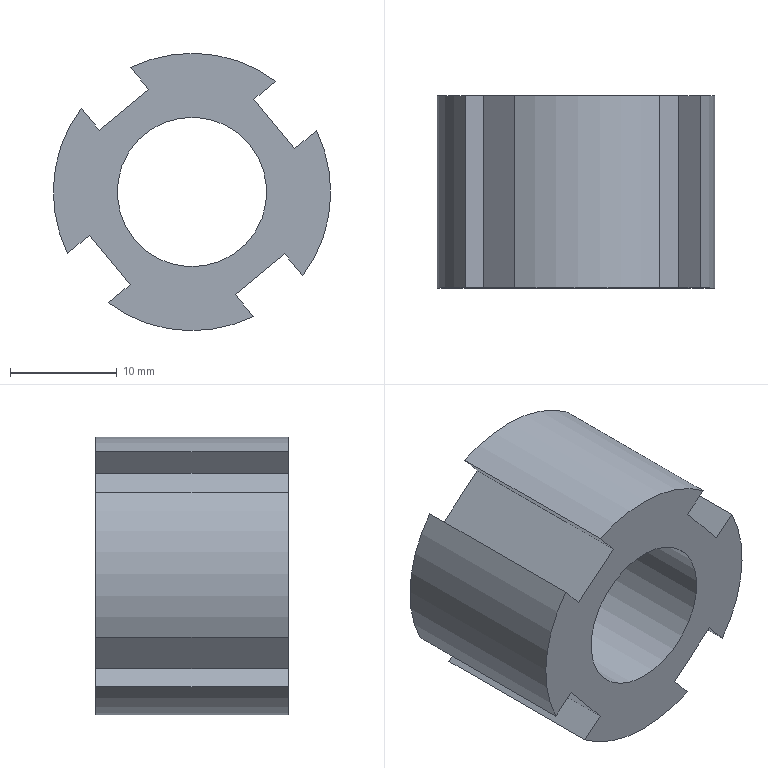Component | SolidWorks | TurntableFixingNut-1 | 1 solid | 20 faces | box 26 x 18 x 26 mm | volume 5540 mm3 | plane 14 | cylinder 6 | commonest cylinder face diameters 26 x4 14 x2
STEP:
#1=COLOUR_RGB('',0.7922,0.8196,0.9333);
#2=FILL_AREA_STYLE_COLOUR('',#1);
#3=FILL_AREA_STYLE('',(#2));
#4=SURFACE_STYLE_FILL_AREA(#3);
#5=SURFACE_SIDE_STYLE('',(#4));
#6=SURFACE_STYLE_USAGE(.BOTH.,#5);
#7=PRESENTATION_STYLE_ASSIGNMENT((#6));
#8=CARTESIAN_POINT('',(-4.58,21.141,7.611));
#9=VERTEX_POINT('',#8);
#10=CARTESIAN_POINT('',(-4.155,21.141,7.963));
#11=VERTEX_POINT('',#10);
#12=CARTESIAN_POINT('',(-4.368,21.141,7.787));
#13=DIRECTION('',(0.,1.,0.));
#14=DIRECTION('',(0.7706,0.,0.6373));
#15=AXIS2_PLACEMENT_3D('',#12,#13,#14);
#16=CIRCLE('',#15,0.2756);
#17=EDGE_CURVE('',#9,#11,#16,.T.);
#18=ORIENTED_EDGE('',*,*,#17,.F.);
#19=CARTESIAN_POINT('',(-4.58,21.85,7.611));
#20=VERTEX_POINT('',#19);
#21=CARTESIAN_POINT('',(-4.58,21.85,7.611));
#22=DIRECTION('',(0.,1.,0.));
#23=VECTOR('',#22,39.37);
#24=LINE('',#21,#23);
#25=EDGE_CURVE('',#9,#20,#24,.T.);
#26=ORIENTED_EDGE('',*,*,#25,.T.);
#27=CARTESIAN_POINT('',(-4.155,21.85,7.963));
#28=VERTEX_POINT('',#27);
#29=CARTESIAN_POINT('',(-4.368,21.85,7.787));
#30=DIRECTION('',(0.,1.,0.));
#31=DIRECTION('',(0.7706,0.,0.6373));
#32=AXIS2_PLACEMENT_3D('',#29,#30,#31);
#33=CIRCLE('',#32,0.2756);
#34=EDGE_CURVE('',#20,#28,#33,.T.);
#35=ORIENTED_EDGE('',*,*,#34,.T.);
#36=CARTESIAN_POINT('',(-4.155,21.85,7.963));
#37=DIRECTION('',(0.,1.,0.));
#38=VECTOR('',#37,39.37);
#39=LINE('',#36,#38);
#40=EDGE_CURVE('',#11,#28,#39,.T.);
#41=ORIENTED_EDGE('',*,*,#40,.F.);
#42=EDGE_LOOP('',(#18,#26,#35,#41));
#43=FACE_OUTER_BOUND('',#42,.T.);
#44=CARTESIAN_POINT('',(-4.368,21.85,7.787));
#45=DIRECTION('',(0.,1.,0.));
#46=DIRECTION('',(0.7706,0.,0.6373));
#47=AXIS2_PLACEMENT_3D('',#44,#45,#46);
#48=CYLINDRICAL_SURFACE('',#47,0.2756);
#49=ADVANCED_FACE('',(#43),#48,.F.);
#50=CARTESIAN_POINT('',(-4.827,21.141,7.561));
#51=VERTEX_POINT('',#50);
#52=CARTESIAN_POINT('',(-4.776,21.141,8.095));
#53=VERTEX_POINT('',#52);
#54=CARTESIAN_POINT('',(-4.368,21.141,7.787));
#55=DIRECTION('',(0.,1.,0.));
#56=DIRECTION('',(0.7706,0.,0.6373));
#57=AXIS2_PLACEMENT_3D('',#54,#55,#56);
#58=CIRCLE('',#57,0.5118);
#59=EDGE_CURVE('',#51,#53,#58,.T.);
#60=ORIENTED_EDGE('',*,*,#59,.T.);
#61=CARTESIAN_POINT('',(-4.776,21.85,8.095));
#62=VERTEX_POINT('',#61);
#63=CARTESIAN_POINT('',(-4.776,21.85,8.095));
#64=DIRECTION('',(0.,-1.,0.));
#65=VECTOR('',#64,39.37);
#66=LINE('',#63,#65);
#67=EDGE_CURVE('',#62,#53,#66,.T.);
#68=ORIENTED_EDGE('',*,*,#67,.F.);
#69=CARTESIAN_POINT('',(-4.827,21.85,7.561));
#70=VERTEX_POINT('',#69);
#71=CARTESIAN_POINT('',(-4.368,21.85,7.787));
#72=DIRECTION('',(0.,1.,0.));
#73=DIRECTION('',(0.7706,0.,0.6373));
#74=AXIS2_PLACEMENT_3D('',#71,#72,#73);
#75=CIRCLE('',#74,0.5118);
#76=EDGE_CURVE('',#70,#62,#75,.T.);
#77=ORIENTED_EDGE('',*,*,#76,.F.);
#78=CARTESIAN_POINT('',(-4.827,21.85,7.561));
#79=DIRECTION('',(0.,-1.,0.));
#80=VECTOR('',#79,39.37);
#81=LINE('',#78,#80);
#82=EDGE_CURVE('',#70,#51,#81,.T.);
#83=ORIENTED_EDGE('',*,*,#82,.T.);
#84=EDGE_LOOP('',(#60,#68,#77,#83));
#85=FACE_OUTER_BOUND('',#84,.T.);
#86=CARTESIAN_POINT('',(-4.368,21.85,7.787));
#87=DIRECTION('',(0.,-1.,0.));
#88=DIRECTION('',(-0.7706,0.,-0.6373));
#89=AXIS2_PLACEMENT_3D('',#86,#87,#88);
#90=CYLINDRICAL_SURFACE('',#89,0.5118);
#91=ADVANCED_FACE('',(#85),#90,.T.);
#92=CARTESIAN_POINT('',(-4.71,21.141,8.015));
#93=VERTEX_POINT('',#92);
#94=CARTESIAN_POINT('',(-4.776,21.141,8.095));
#95=DIRECTION('',(0.6373,0.,-0.7706));
#96=VECTOR('',#95,39.37);
#97=LINE('',#94,#96);
#98=EDGE_CURVE('',#53,#93,#97,.T.);
#99=ORIENTED_EDGE('',*,*,#98,.T.);
#100=CARTESIAN_POINT('',(-4.71,21.85,8.015));
#101=VERTEX_POINT('',#100);
#102=CARTESIAN_POINT('',(-4.71,21.85,8.015));
#103=DIRECTION('',(0.,-1.,0.));
#104=VECTOR('',#103,39.37);
#105=LINE('',#102,#104);
#106=EDGE_CURVE('',#101,#93,#105,.T.);
#107=ORIENTED_EDGE('',*,*,#106,.F.);
#108=CARTESIAN_POINT('',(-4.776,21.85,8.095));
#109=DIRECTION('',(0.6373,0.,-0.7706));
#110=VECTOR('',#109,39.37);
#111=LINE('',#108,#110);
#112=EDGE_CURVE('',#62,#101,#111,.T.);
#113=ORIENTED_EDGE('',*,*,#112,.F.);
#114=ORIENTED_EDGE('',*,*,#67,.T.);
#115=EDGE_LOOP('',(#99,#107,#113,#114));
#116=FACE_OUTER_BOUND('',#115,.T.);
#117=CARTESIAN_POINT('',(-4.776,21.85,8.095));
#118=DIRECTION('',(-0.7706,0.,-0.6373));
#119=DIRECTION('',(-0.6373,0.,0.7706));
#120=AXIS2_PLACEMENT_3D('',#117,#118,#119);
#121=PLANE('',#120);
#122=ADVANCED_FACE('',(#116),#121,.F.);
#123=CARTESIAN_POINT('',(-4.528,21.141,8.166));
#124=VERTEX_POINT('',#123);
#125=CARTESIAN_POINT('',(-4.528,21.141,8.166));
#126=DIRECTION('',(0.7706,0.,0.6373));
#127=VECTOR('',#126,39.37);
#128=LINE('',#125,#127);
#129=EDGE_CURVE('',#93,#124,#128,.T.);
#130=ORIENTED_EDGE('',*,*,#129,.T.);
#131=CARTESIAN_POINT('',(-4.528,21.85,8.166));
#132=VERTEX_POINT('',#131);
#133=CARTESIAN_POINT('',(-4.528,21.85,8.166));
#134=DIRECTION('',(0.,-1.,0.));
#135=VECTOR('',#134,39.37);
#136=LINE('',#133,#135);
#137=EDGE_CURVE('',#132,#124,#136,.T.);
#138=ORIENTED_EDGE('',*,*,#137,.F.);
#139=CARTESIAN_POINT('',(-4.528,21.85,8.166));
#140=DIRECTION('',(0.7706,0.,0.6373));
#141=VECTOR('',#140,39.37);
#142=LINE('',#139,#141);
#143=EDGE_CURVE('',#101,#132,#142,.T.);
#144=ORIENTED_EDGE('',*,*,#143,.F.);
#145=ORIENTED_EDGE('',*,*,#106,.T.);
#146=EDGE_LOOP('',(#130,#138,#144,#145));
#147=FACE_OUTER_BOUND('',#146,.T.);
#148=CARTESIAN_POINT('',(-4.528,21.85,8.166));
#149=DIRECTION('',(0.6373,0.,-0.7706));
#150=DIRECTION('',(-0.7706,0.,-0.6373));
#151=AXIS2_PLACEMENT_3D('',#148,#149,#150);
#152=PLANE('',#151);
#153=ADVANCED_FACE('',(#147),#152,.F.);
#154=CARTESIAN_POINT('',(-4.594,21.141,8.246));
#155=VERTEX_POINT('',#154);
#156=CARTESIAN_POINT('',(-4.594,21.141,8.246));
#157=DIRECTION('',(-0.6373,0.,0.7706));
#158=VECTOR('',#157,39.37);
#159=LINE('',#156,#158);
#160=EDGE_CURVE('',#124,#155,#159,.T.);
#161=ORIENTED_EDGE('',*,*,#160,.T.);
#162=CARTESIAN_POINT('',(-4.594,21.85,8.246));
#163=VERTEX_POINT('',#162);
#164=CARTESIAN_POINT('',(-4.594,21.85,8.246));
#165=DIRECTION('',(0.,-1.,0.));
#166=VECTOR('',#165,39.37);
#167=LINE('',#164,#166);
#168=EDGE_CURVE('',#163,#155,#167,.T.);
#169=ORIENTED_EDGE('',*,*,#168,.F.);
#170=CARTESIAN_POINT('',(-4.594,21.85,8.246));
#171=DIRECTION('',(-0.6373,0.,0.7706));
#172=VECTOR('',#171,39.37);
#173=LINE('',#170,#172);
#174=EDGE_CURVE('',#132,#163,#173,.T.);
#175=ORIENTED_EDGE('',*,*,#174,.F.);
#176=ORIENTED_EDGE('',*,*,#137,.T.);
#177=EDGE_LOOP('',(#161,#169,#175,#176));
#178=FACE_OUTER_BOUND('',#177,.T.);
#179=CARTESIAN_POINT('',(-4.594,21.85,8.246));
#180=DIRECTION('',(0.7706,0.,0.6373));
#181=DIRECTION('',(0.6373,0.,-0.7706));
#182=AXIS2_PLACEMENT_3D('',#179,#180,#181);
#183=PLANE('',#182);
#184=ADVANCED_FACE('',(#178),#183,.F.);
#185=CARTESIAN_POINT('',(-4.059,21.141,8.195));
#186=VERTEX_POINT('',#185);
#187=CARTESIAN_POINT('',(-4.368,21.141,7.787));
#188=DIRECTION('',(0.,1.,0.));
#189=DIRECTION('',(0.7706,0.,0.6373));
#190=AXIS2_PLACEMENT_3D('',#187,#188,#189);
#191=CIRCLE('',#190,0.5118);
#192=EDGE_CURVE('',#155,#186,#191,.T.);
#193=ORIENTED_EDGE('',*,*,#192,.T.);
#194=CARTESIAN_POINT('',(-4.059,21.85,8.195));
#195=VERTEX_POINT('',#194);
#196=CARTESIAN_POINT('',(-4.059,21.85,8.195));
#197=DIRECTION('',(0.,-1.,0.));
#198=VECTOR('',#197,39.37);
#199=LINE('',#196,#198);
#200=EDGE_CURVE('',#195,#186,#199,.T.);
#201=ORIENTED_EDGE('',*,*,#200,.F.);
#202=CARTESIAN_POINT('',(-4.368,21.85,7.787));
#203=DIRECTION('',(0.,1.,0.));
#204=DIRECTION('',(0.7706,0.,0.6373));
#205=AXIS2_PLACEMENT_3D('',#202,#203,#204);
#206=CIRCLE('',#205,0.5118);
#207=EDGE_CURVE('',#163,#195,#206,.T.);
#208=ORIENTED_EDGE('',*,*,#207,.F.);
#209=ORIENTED_EDGE('',*,*,#168,.T.);
#210=EDGE_LOOP('',(#193,#201,#208,#209));
#211=FACE_OUTER_BOUND('',#210,.T.);
#212=CARTESIAN_POINT('',(-4.368,21.85,7.787));
#213=DIRECTION('',(0.,-1.,0.));
#214=DIRECTION('',(-0.7706,0.,-0.6373));
#215=AXIS2_PLACEMENT_3D('',#212,#213,#214);
#216=CYLINDRICAL_SURFACE('',#215,0.5118);
#217=ADVANCED_FACE('',(#211),#216,.T.);
#218=CARTESIAN_POINT('',(-4.14,21.141,8.129));
#219=VERTEX_POINT('',#218);
#220=CARTESIAN_POINT('',(-4.059,21.141,8.195));
#221=DIRECTION('',(-0.7706,0.,-0.6373));
#222=VECTOR('',#221,39.37);
#223=LINE('',#220,#222);
#224=EDGE_CURVE('',#186,#219,#223,.T.);
#225=ORIENTED_EDGE('',*,*,#224,.T.);
#226=CARTESIAN_POINT('',(-4.14,21.85,8.129));
#227=VERTEX_POINT('',#226);
#228=CARTESIAN_POINT('',(-4.14,21.85,8.129));
#229=DIRECTION('',(0.,-1.,0.));
#230=VECTOR('',#229,39.37);
#231=LINE('',#228,#230);
#232=EDGE_CURVE('',#227,#219,#231,.T.);
#233=ORIENTED_EDGE('',*,*,#232,.F.);
#234=CARTESIAN_POINT('',(-4.059,21.85,8.195));
#235=DIRECTION('',(-0.7706,0.,-0.6373));
#236=VECTOR('',#235,39.37);
#237=LINE('',#234,#236);
#238=EDGE_CURVE('',#195,#227,#237,.T.);
#239=ORIENTED_EDGE('',*,*,#238,.F.);
#240=ORIENTED_EDGE('',*,*,#200,.T.);
#241=EDGE_LOOP('',(#225,#233,#239,#240));
#242=FACE_OUTER_BOUND('',#241,.T.);
#243=CARTESIAN_POINT('',(-4.059,21.85,8.195));
#244=DIRECTION('',(-0.6373,0.,0.7706));
#245=DIRECTION('',(0.7706,0.,0.6373));
#246=AXIS2_PLACEMENT_3D('',#243,#244,#245);
#247=PLANE('',#246);
#248=ADVANCED_FACE('',(#242),#247,.F.);
#249=CARTESIAN_POINT('',(-3.989,21.141,7.947));
#250=VERTEX_POINT('',#249);
#251=CARTESIAN_POINT('',(-3.989,21.141,7.947));
#252=DIRECTION('',(0.6373,0.,-0.7706));
#253=VECTOR('',#252,39.37);
#254=LINE('',#251,#253);
#255=EDGE_CURVE('',#219,#250,#254,.T.);
#256=ORIENTED_EDGE('',*,*,#255,.T.);
#257=CARTESIAN_POINT('',(-3.989,21.85,7.947));
#258=VERTEX_POINT('',#257);
#259=CARTESIAN_POINT('',(-3.989,21.85,7.947));
#260=DIRECTION('',(0.,-1.,0.));
#261=VECTOR('',#260,39.37);
#262=LINE('',#259,#261);
#263=EDGE_CURVE('',#258,#250,#262,.T.);
#264=ORIENTED_EDGE('',*,*,#263,.F.);
#265=CARTESIAN_POINT('',(-3.989,21.85,7.947));
#266=DIRECTION('',(0.6373,0.,-0.7706));
#267=VECTOR('',#266,39.37);
#268=LINE('',#265,#267);
#269=EDGE_CURVE('',#227,#258,#268,.T.);
#270=ORIENTED_EDGE('',*,*,#269,.F.);
#271=ORIENTED_EDGE('',*,*,#232,.T.);
#272=EDGE_LOOP('',(#256,#264,#270,#271));
#273=FACE_OUTER_BOUND('',#272,.T.);
#274=CARTESIAN_POINT('',(-3.989,21.85,7.947));
#275=DIRECTION('',(-0.7706,0.,-0.6373));
#276=DIRECTION('',(-0.6373,0.,0.7706));
#277=AXIS2_PLACEMENT_3D('',#274,#275,#276);
#278=PLANE('',#277);
#279=ADVANCED_FACE('',(#273),#278,.F.);
#280=CARTESIAN_POINT('',(-3.909,21.141,8.013));
#281=VERTEX_POINT('',#280);
#282=CARTESIAN_POINT('',(-3.909,21.141,8.013));
#283=DIRECTION('',(0.7706,0.,0.6373));
#284=VECTOR('',#283,39.37);
#285=LINE('',#282,#284);
#286=EDGE_CURVE('',#250,#281,#285,.T.);
#287=ORIENTED_EDGE('',*,*,#286,.T.);
#288=CARTESIAN_POINT('',(-3.909,21.85,8.013));
#289=VERTEX_POINT('',#288);
#290=CARTESIAN_POINT('',(-3.909,21.85,8.013));
#291=DIRECTION('',(0.,-1.,0.));
#292=VECTOR('',#291,39.37);
#293=LINE('',#290,#292);
#294=EDGE_CURVE('',#289,#281,#293,.T.);
#295=ORIENTED_EDGE('',*,*,#294,.F.);
#296=CARTESIAN_POINT('',(-3.909,21.85,8.013));
#297=DIRECTION('',(0.7706,0.,0.6373));
#298=VECTOR('',#297,39.37);
#299=LINE('',#296,#298);
#300=EDGE_CURVE('',#258,#289,#299,.T.);
#301=ORIENTED_EDGE('',*,*,#300,.F.);
#302=ORIENTED_EDGE('',*,*,#263,.T.);
#303=EDGE_LOOP('',(#287,#295,#301,#302));
#304=FACE_OUTER_BOUND('',#303,.T.);
#305=CARTESIAN_POINT('',(-3.909,21.85,8.013));
#306=DIRECTION('',(0.6373,0.,-0.7706));
#307=DIRECTION('',(-0.7706,0.,-0.6373));
#308=AXIS2_PLACEMENT_3D('',#305,#306,#307);
#309=PLANE('',#308);
#310=ADVANCED_FACE('',(#304),#309,.F.);
#311=CARTESIAN_POINT('',(-3.959,21.141,7.478));
#312=VERTEX_POINT('',#311);
#313=CARTESIAN_POINT('',(-4.368,21.141,7.787));
#314=DIRECTION('',(0.,1.,0.));
#315=DIRECTION('',(0.7706,0.,0.6373));
#316=AXIS2_PLACEMENT_3D('',#313,#314,#315);
#317=CIRCLE('',#316,0.5118);
#318=EDGE_CURVE('',#281,#312,#317,.T.);
#319=ORIENTED_EDGE('',*,*,#318,.T.);
#320=CARTESIAN_POINT('',(-3.959,21.85,7.478));
#321=VERTEX_POINT('',#320);
#322=CARTESIAN_POINT('',(-3.959,21.85,7.478));
#323=DIRECTION('',(0.,-1.,0.));
#324=VECTOR('',#323,39.37);
#325=LINE('',#322,#324);
#326=EDGE_CURVE('',#321,#312,#325,.T.);
#327=ORIENTED_EDGE('',*,*,#326,.F.);
#328=CARTESIAN_POINT('',(-4.368,21.85,7.787));
#329=DIRECTION('',(0.,1.,0.));
#330=DIRECTION('',(0.7706,0.,0.6373));
#331=AXIS2_PLACEMENT_3D('',#328,#329,#330);
#332=CIRCLE('',#331,0.5118);
#333=EDGE_CURVE('',#289,#321,#332,.T.);
#334=ORIENTED_EDGE('',*,*,#333,.F.);
#335=ORIENTED_EDGE('',*,*,#294,.T.);
#336=EDGE_LOOP('',(#319,#327,#334,#335));
#337=FACE_OUTER_BOUND('',#336,.T.);
#338=CARTESIAN_POINT('',(-4.368,21.85,7.787));
#339=DIRECTION('',(0.,-1.,0.));
#340=DIRECTION('',(-0.7706,0.,-0.6373));
#341=AXIS2_PLACEMENT_3D('',#338,#339,#340);
#342=CYLINDRICAL_SURFACE('',#341,0.5118);
#343=ADVANCED_FACE('',(#337),#342,.T.);
#344=CARTESIAN_POINT('',(-4.026,21.141,7.559));
#345=VERTEX_POINT('',#344);
#346=CARTESIAN_POINT('',(-3.959,21.141,7.478));
#347=DIRECTION('',(-0.6373,0.,0.7706));
#348=VECTOR('',#347,39.37);
#349=LINE('',#346,#348);
#350=EDGE_CURVE('',#312,#345,#349,.T.);
#351=ORIENTED_EDGE('',*,*,#350,.T.);
#352=CARTESIAN_POINT('',(-4.026,21.85,7.559));
#353=VERTEX_POINT('',#352);
#354=CARTESIAN_POINT('',(-4.026,21.85,7.559));
#355=DIRECTION('',(0.,-1.,0.));
#356=VECTOR('',#355,39.37);
#357=LINE('',#354,#356);
#358=EDGE_CURVE('',#353,#345,#357,.T.);
#359=ORIENTED_EDGE('',*,*,#358,.F.);
#360=CARTESIAN_POINT('',(-3.959,21.85,7.478));
#361=DIRECTION('',(-0.6373,0.,0.7706));
#362=VECTOR('',#361,39.37);
#363=LINE('',#360,#362);
#364=EDGE_CURVE('',#321,#353,#363,.T.);
#365=ORIENTED_EDGE('',*,*,#364,.F.);
#366=ORIENTED_EDGE('',*,*,#326,.T.);
#367=EDGE_LOOP('',(#351,#359,#365,#366));
#368=FACE_OUTER_BOUND('',#367,.T.);
#369=CARTESIAN_POINT('',(-3.959,21.85,7.478));
#370=DIRECTION('',(0.7706,0.,0.6373));
#371=DIRECTION('',(0.6373,0.,-0.7706));
#372=AXIS2_PLACEMENT_3D('',#369,#370,#371);
#373=PLANE('',#372);
#374=ADVANCED_FACE('',(#368),#373,.F.);
#375=CARTESIAN_POINT('',(-4.208,21.141,7.408));
#376=VERTEX_POINT('',#375);
#377=CARTESIAN_POINT('',(-4.208,21.141,7.408));
#378=DIRECTION('',(-0.7706,0.,-0.6373));
#379=VECTOR('',#378,39.37);
#380=LINE('',#377,#379);
#381=EDGE_CURVE('',#345,#376,#380,.T.);
#382=ORIENTED_EDGE('',*,*,#381,.T.);
#383=CARTESIAN_POINT('',(-4.208,21.85,7.408));
#384=VERTEX_POINT('',#383);
#385=CARTESIAN_POINT('',(-4.208,21.85,7.408));
#386=DIRECTION('',(0.,-1.,0.));
#387=VECTOR('',#386,39.37);
#388=LINE('',#385,#387);
#389=EDGE_CURVE('',#384,#376,#388,.T.);
#390=ORIENTED_EDGE('',*,*,#389,.F.);
#391=CARTESIAN_POINT('',(-4.208,21.85,7.408));
#392=DIRECTION('',(-0.7706,0.,-0.6373));
#393=VECTOR('',#392,39.37);
#394=LINE('',#391,#393);
#395=EDGE_CURVE('',#353,#384,#394,.T.);
#396=ORIENTED_EDGE('',*,*,#395,.F.);
#397=ORIENTED_EDGE('',*,*,#358,.T.);
#398=EDGE_LOOP('',(#382,#390,#396,#397));
#399=FACE_OUTER_BOUND('',#398,.T.);
#400=CARTESIAN_POINT('',(-4.208,21.85,7.408));
#401=DIRECTION('',(-0.6373,0.,0.7706));
#402=DIRECTION('',(0.7706,0.,0.6373));
#403=AXIS2_PLACEMENT_3D('',#400,#401,#402);
#404=PLANE('',#403);
#405=ADVANCED_FACE('',(#399),#404,.F.);
#406=CARTESIAN_POINT('',(-4.142,21.141,7.328));
#407=VERTEX_POINT('',#406);
#408=CARTESIAN_POINT('',(-4.142,21.141,7.328));
#409=DIRECTION('',(0.6373,0.,-0.7706));
#410=VECTOR('',#409,39.37);
#411=LINE('',#408,#410);
#412=EDGE_CURVE('',#376,#407,#411,.T.);
#413=ORIENTED_EDGE('',*,*,#412,.T.);
#414=CARTESIAN_POINT('',(-4.142,21.85,7.328));
#415=VERTEX_POINT('',#414);
#416=CARTESIAN_POINT('',(-4.142,21.85,7.328));
#417=DIRECTION('',(0.,-1.,0.));
#418=VECTOR('',#417,39.37);
#419=LINE('',#416,#418);
#420=EDGE_CURVE('',#415,#407,#419,.T.);
#421=ORIENTED_EDGE('',*,*,#420,.F.);
#422=CARTESIAN_POINT('',(-4.142,21.85,7.328));
#423=DIRECTION('',(0.6373,0.,-0.7706));
#424=VECTOR('',#423,39.37);
#425=LINE('',#422,#424);
#426=EDGE_CURVE('',#384,#415,#425,.T.);
#427=ORIENTED_EDGE('',*,*,#426,.F.);
#428=ORIENTED_EDGE('',*,*,#389,.T.);
#429=EDGE_LOOP('',(#413,#421,#427,#428));
#430=FACE_OUTER_BOUND('',#429,.T.);
#431=CARTESIAN_POINT('',(-4.142,21.85,7.328));
#432=DIRECTION('',(-0.7706,0.,-0.6373));
#433=DIRECTION('',(-0.6373,0.,0.7706));
#434=AXIS2_PLACEMENT_3D('',#431,#432,#433);
#435=PLANE('',#434);
#436=ADVANCED_FACE('',(#430),#435,.F.);
#437=CARTESIAN_POINT('',(-4.676,21.141,7.379));
#438=VERTEX_POINT('',#437);
#439=CARTESIAN_POINT('',(-4.368,21.141,7.787));
#440=DIRECTION('',(0.,1.,0.));
#441=DIRECTION('',(0.7706,0.,0.6373));
#442=AXIS2_PLACEMENT_3D('',#439,#440,#441);
#443=CIRCLE('',#442,0.5118);
#444=EDGE_CURVE('',#407,#438,#443,.T.);
#445=ORIENTED_EDGE('',*,*,#444,.T.);
#446=CARTESIAN_POINT('',(-4.676,21.85,7.379));
#447=VERTEX_POINT('',#446);
#448=CARTESIAN_POINT('',(-4.676,21.85,7.379));
#449=DIRECTION('',(0.,-1.,0.));
#450=VECTOR('',#449,39.37);
#451=LINE('',#448,#450);
#452=EDGE_CURVE('',#447,#438,#451,.T.);
#453=ORIENTED_EDGE('',*,*,#452,.F.);
#454=CARTESIAN_POINT('',(-4.368,21.85,7.787));
#455=DIRECTION('',(0.,1.,0.));
#456=DIRECTION('',(0.7706,0.,0.6373));
#457=AXIS2_PLACEMENT_3D('',#454,#455,#456);
#458=CIRCLE('',#457,0.5118);
#459=EDGE_CURVE('',#415,#447,#458,.T.);
#460=ORIENTED_EDGE('',*,*,#459,.F.);
#461=ORIENTED_EDGE('',*,*,#420,.T.);
#462=EDGE_LOOP('',(#445,#453,#460,#461));
#463=FACE_OUTER_BOUND('',#462,.T.);
#464=CARTESIAN_POINT('',(-4.368,21.85,7.787));
#465=DIRECTION('',(0.,-1.,0.));
#466=DIRECTION('',(-0.7706,0.,-0.6373));
#467=AXIS2_PLACEMENT_3D('',#464,#465,#466);
#468=CYLINDRICAL_SURFACE('',#467,0.5118);
#469=ADVANCED_FACE('',(#463),#468,.T.);
#470=CARTESIAN_POINT('',(-4.596,21.141,7.445));
#471=VERTEX_POINT('',#470);
#472=CARTESIAN_POINT('',(-4.676,21.141,7.379));
#473=DIRECTION('',(0.7706,0.,0.6373));
#474=VECTOR('',#473,39.37);
#475=LINE('',#472,#474);
#476=EDGE_CURVE('',#438,#471,#475,.T.);
#477=ORIENTED_EDGE('',*,*,#476,.T.);
#478=CARTESIAN_POINT('',(-4.596,21.85,7.445));
#479=VERTEX_POINT('',#478);
#480=CARTESIAN_POINT('',(-4.596,21.85,7.445));
#481=DIRECTION('',(0.,-1.,0.));
#482=VECTOR('',#481,39.37);
#483=LINE('',#480,#482);
#484=EDGE_CURVE('',#479,#471,#483,.T.);
#485=ORIENTED_EDGE('',*,*,#484,.F.);
#486=CARTESIAN_POINT('',(-4.676,21.85,7.379));
#487=DIRECTION('',(0.7706,0.,0.6373));
#488=VECTOR('',#487,39.37);
#489=LINE('',#486,#488);
#490=EDGE_CURVE('',#447,#479,#489,.T.);
#491=ORIENTED_EDGE('',*,*,#490,.F.);
#492=ORIENTED_EDGE('',*,*,#452,.T.);
#493=EDGE_LOOP('',(#477,#485,#491,#492));
#494=FACE_OUTER_BOUND('',#493,.T.);
#495=CARTESIAN_POINT('',(-4.676,21.85,7.379));
#496=DIRECTION('',(0.6373,0.,-0.7706));
#497=DIRECTION('',(-0.7706,0.,-0.6373));
#498=AXIS2_PLACEMENT_3D('',#495,#496,#497);
#499=PLANE('',#498);
#500=ADVANCED_FACE('',(#494),#499,.F.);
#501=CARTESIAN_POINT('',(-4.747,21.141,7.627));
#502=VERTEX_POINT('',#501);
#503=CARTESIAN_POINT('',(-4.747,21.141,7.627));
#504=DIRECTION('',(-0.6373,0.,0.7706));
#505=VECTOR('',#504,39.37);
#506=LINE('',#503,#505);
#507=EDGE_CURVE('',#471,#502,#506,.T.);
#508=ORIENTED_EDGE('',*,*,#507,.T.);
#509=CARTESIAN_POINT('',(-4.747,21.85,7.627));
#510=VERTEX_POINT('',#509);
#511=CARTESIAN_POINT('',(-4.747,21.85,7.627));
#512=DIRECTION('',(0.,-1.,0.));
#513=VECTOR('',#512,39.37);
#514=LINE('',#511,#513);
#515=EDGE_CURVE('',#510,#502,#514,.T.);
#516=ORIENTED_EDGE('',*,*,#515,.F.);
#517=CARTESIAN_POINT('',(-4.747,21.85,7.627));
#518=DIRECTION('',(-0.6373,0.,0.7706));
#519=VECTOR('',#518,39.37);
#520=LINE('',#517,#519);
#521=EDGE_CURVE('',#479,#510,#520,.T.);
#522=ORIENTED_EDGE('',*,*,#521,.F.);
#523=ORIENTED_EDGE('',*,*,#484,.T.);
#524=EDGE_LOOP('',(#508,#516,#522,#523));
#525=FACE_OUTER_BOUND('',#524,.T.);
#526=CARTESIAN_POINT('',(-4.747,21.85,7.627));
#527=DIRECTION('',(0.7706,0.,0.6373));
#528=DIRECTION('',(0.6373,0.,-0.7706));
#529=AXIS2_PLACEMENT_3D('',#526,#527,#528);
#530=PLANE('',#529);
#531=ADVANCED_FACE('',(#525),#530,.F.);
#532=CARTESIAN_POINT('',(-4.827,21.141,7.561));
#533=DIRECTION('',(-0.7706,0.,-0.6373));
#534=VECTOR('',#533,39.37);
#535=LINE('',#532,#534);
#536=EDGE_CURVE('',#502,#51,#535,.T.);
#537=ORIENTED_EDGE('',*,*,#536,.T.);
#538=ORIENTED_EDGE('',*,*,#82,.F.);
#539=CARTESIAN_POINT('',(-4.827,21.85,7.561));
#540=DIRECTION('',(-0.7706,0.,-0.6373));
#541=VECTOR('',#540,39.37);
#542=LINE('',#539,#541);
#543=EDGE_CURVE('',#510,#70,#542,.T.);
#544=ORIENTED_EDGE('',*,*,#543,.F.);
#545=ORIENTED_EDGE('',*,*,#515,.T.);
#546=EDGE_LOOP('',(#537,#538,#544,#545));
#547=FACE_OUTER_BOUND('',#546,.T.);
#548=CARTESIAN_POINT('',(-4.827,21.85,7.561));
#549=DIRECTION('',(-0.6373,0.,0.7706));
#550=DIRECTION('',(0.7706,0.,0.6373));
#551=AXIS2_PLACEMENT_3D('',#548,#549,#550);
#552=PLANE('',#551);
#553=ADVANCED_FACE('',(#547),#552,.F.);
#554=CARTESIAN_POINT('',(-4.368,21.85,7.787));
#555=DIRECTION('',(0.,1.,0.));
#556=DIRECTION('',(0.7706,0.,0.6373));
#557=AXIS2_PLACEMENT_3D('',#554,#555,#556);
#558=CIRCLE('',#557,0.2756);
#559=EDGE_CURVE('',#28,#20,#558,.T.);
#560=ORIENTED_EDGE('',*,*,#559,.F.);
#561=ORIENTED_EDGE('',*,*,#34,.F.);
#562=EDGE_LOOP('',(#560,#561));
#563=FACE_BOUND('',#562,.T.);
#564=ORIENTED_EDGE('',*,*,#76,.T.);
#565=ORIENTED_EDGE('',*,*,#112,.T.);
#566=ORIENTED_EDGE('',*,*,#143,.T.);
#567=ORIENTED_EDGE('',*,*,#174,.T.);
#568=ORIENTED_EDGE('',*,*,#207,.T.);
#569=ORIENTED_EDGE('',*,*,#238,.T.);
#570=ORIENTED_EDGE('',*,*,#269,.T.);
#571=ORIENTED_EDGE('',*,*,#300,.T.);
#572=ORIENTED_EDGE('',*,*,#333,.T.);
#573=ORIENTED_EDGE('',*,*,#364,.T.);
#574=ORIENTED_EDGE('',*,*,#395,.T.);
#575=ORIENTED_EDGE('',*,*,#426,.T.);
#576=ORIENTED_EDGE('',*,*,#459,.T.);
#577=ORIENTED_EDGE('',*,*,#490,.T.);
#578=ORIENTED_EDGE('',*,*,#521,.T.);
#579=ORIENTED_EDGE('',*,*,#543,.T.);
#580=EDGE_LOOP('',(#564,#565,#566,#567,#568,#569,#570,#571,#572,#573,#574,#575,#576,#577,#578,#579));
#581=FACE_OUTER_BOUND('',#580,.T.);
#582=CARTESIAN_POINT('',(-4.368,21.85,7.787));
#583=DIRECTION('',(0.,1.,0.));
#584=DIRECTION('',(0.7706,0.,0.6373));
#585=AXIS2_PLACEMENT_3D('',#582,#583,#584);
#586=PLANE('',#585);
#587=ADVANCED_FACE('',(#563,#581),#586,.T.);
#588=CARTESIAN_POINT('',(-4.368,21.141,7.787));
#589=DIRECTION('',(0.,1.,0.));
#590=DIRECTION('',(0.7706,0.,0.6373));
#591=AXIS2_PLACEMENT_3D('',#588,#589,#590);
#592=CIRCLE('',#591,0.2756);
#593=EDGE_CURVE('',#11,#9,#592,.T.);
#594=ORIENTED_EDGE('',*,*,#593,.T.);
#595=ORIENTED_EDGE('',*,*,#17,.T.);
#596=EDGE_LOOP('',(#594,#595));
#597=FACE_BOUND('',#596,.T.);
#598=ORIENTED_EDGE('',*,*,#59,.F.);
#599=ORIENTED_EDGE('',*,*,#536,.F.);
#600=ORIENTED_EDGE('',*,*,#507,.F.);
#601=ORIENTED_EDGE('',*,*,#476,.F.);
#602=ORIENTED_EDGE('',*,*,#444,.F.);
#603=ORIENTED_EDGE('',*,*,#412,.F.);
#604=ORIENTED_EDGE('',*,*,#381,.F.);
#605=ORIENTED_EDGE('',*,*,#350,.F.);
#606=ORIENTED_EDGE('',*,*,#318,.F.);
#607=ORIENTED_EDGE('',*,*,#286,.F.);
#608=ORIENTED_EDGE('',*,*,#255,.F.);
#609=ORIENTED_EDGE('',*,*,#224,.F.);
#610=ORIENTED_EDGE('',*,*,#192,.F.);
#611=ORIENTED_EDGE('',*,*,#160,.F.);
#612=ORIENTED_EDGE('',*,*,#129,.F.);
#613=ORIENTED_EDGE('',*,*,#98,.F.);
#614=EDGE_LOOP('',(#598,#599,#600,#601,#602,#603,#604,#605,#606,#607,#608,#609,#610,#611,#612,#613));
#615=FACE_OUTER_BOUND('',#614,.T.);
#616=CARTESIAN_POINT('',(-4.368,21.141,7.787));
#617=DIRECTION('',(0.,1.,0.));
#618=DIRECTION('',(0.7706,0.,0.6373));
#619=AXIS2_PLACEMENT_3D('',#616,#617,#618);
#620=PLANE('',#619);
#621=ADVANCED_FACE('',(#597,#615),#620,.F.);
#622=ORIENTED_EDGE('',*,*,#25,.F.);
#623=ORIENTED_EDGE('',*,*,#593,.F.);
#624=ORIENTED_EDGE('',*,*,#40,.T.);
#625=ORIENTED_EDGE('',*,*,#559,.T.);
#626=EDGE_LOOP('',(#622,#623,#624,#625));
#627=FACE_OUTER_BOUND('',#626,.T.);
#628=CARTESIAN_POINT('',(-4.368,21.85,7.787));
#629=DIRECTION('',(0.,1.,0.));
#630=DIRECTION('',(0.7706,0.,0.6373));
#631=AXIS2_PLACEMENT_3D('',#628,#629,#630);
#632=CYLINDRICAL_SURFACE('',#631,0.2756);
#633=ADVANCED_FACE('',(#627),#632,.F.);
#634=CLOSED_SHELL('',(#49,#91,#122,#153,#184,#217,#248,#279,#310,#343,#374,#405,#436,#469,#500,#531,#553,#587,#621,#633));
#635=MANIFOLD_SOLID_BREP('',#634);
#636=STYLED_ITEM('',(#7),#635);
#637=(LENGTH_UNIT()NAMED_UNIT(*)SI_UNIT($,.METRE.));
#638=LENGTH_MEASURE_WITH_UNIT(LENGTH_MEASURE(0.0254),#637);
#639=DIMENSIONAL_EXPONENTS(1.,0.,0.,0.,0.,0.,0.);
#640=(CONVERSION_BASED_UNIT('',#638)LENGTH_UNIT()NAMED_UNIT(#639));
#641=UNCERTAINTY_MEASURE_WITH_UNIT(LENGTH_MEASURE(0.00001),#640,'','');
#642=(NAMED_UNIT(*)PLANE_ANGLE_UNIT()SI_UNIT($,.RADIAN.));
#643=(NAMED_UNIT(*)SI_UNIT($,.STERADIAN.)SOLID_ANGLE_UNIT());
#644=(GEOMETRIC_REPRESENTATION_CONTEXT(3)GLOBAL_UNCERTAINTY_ASSIGNED_CONTEXT((#641))GLOBAL_UNIT_ASSIGNED_CONTEXT((#640,#642,#643))REPRESENTATION_CONTEXT('',''));
#645=MECHANICAL_DESIGN_GEOMETRIC_PRESENTATION_REPRESENTATION('',(#636),#644);
#646=CARTESIAN_POINT('',(0.,0.,0.));
#647=DIRECTION('',(0.,0.,1.));
#648=DIRECTION('',(1.,0.,0.));
#649=AXIS2_PLACEMENT_3D('',#646,#647,#648);
#650=(LENGTH_UNIT()NAMED_UNIT(*)SI_UNIT($,.METRE.));
#651=LENGTH_MEASURE_WITH_UNIT(LENGTH_MEASURE(0.0254),#650);
#652=DIMENSIONAL_EXPONENTS(1.,0.,0.,0.,0.,0.,0.);
#653=(CONVERSION_BASED_UNIT('',#651)LENGTH_UNIT()NAMED_UNIT(#652));
#654=UNCERTAINTY_MEASURE_WITH_UNIT(LENGTH_MEASURE(0.00001),#653,'','');
#655=(NAMED_UNIT(*)PLANE_ANGLE_UNIT()SI_UNIT($,.RADIAN.));
#656=(NAMED_UNIT(*)SI_UNIT($,.STERADIAN.)SOLID_ANGLE_UNIT());
#657=(GEOMETRIC_REPRESENTATION_CONTEXT(3)GLOBAL_UNCERTAINTY_ASSIGNED_CONTEXT((#654))GLOBAL_UNIT_ASSIGNED_CONTEXT((#653,#655,#656))REPRESENTATION_CONTEXT('',''));
#658=ADVANCED_BREP_SHAPE_REPRESENTATION('',(#635,#649),#657);
#659=PRESENTATION_LAYER_ASSIGNMENT('','',(#636));